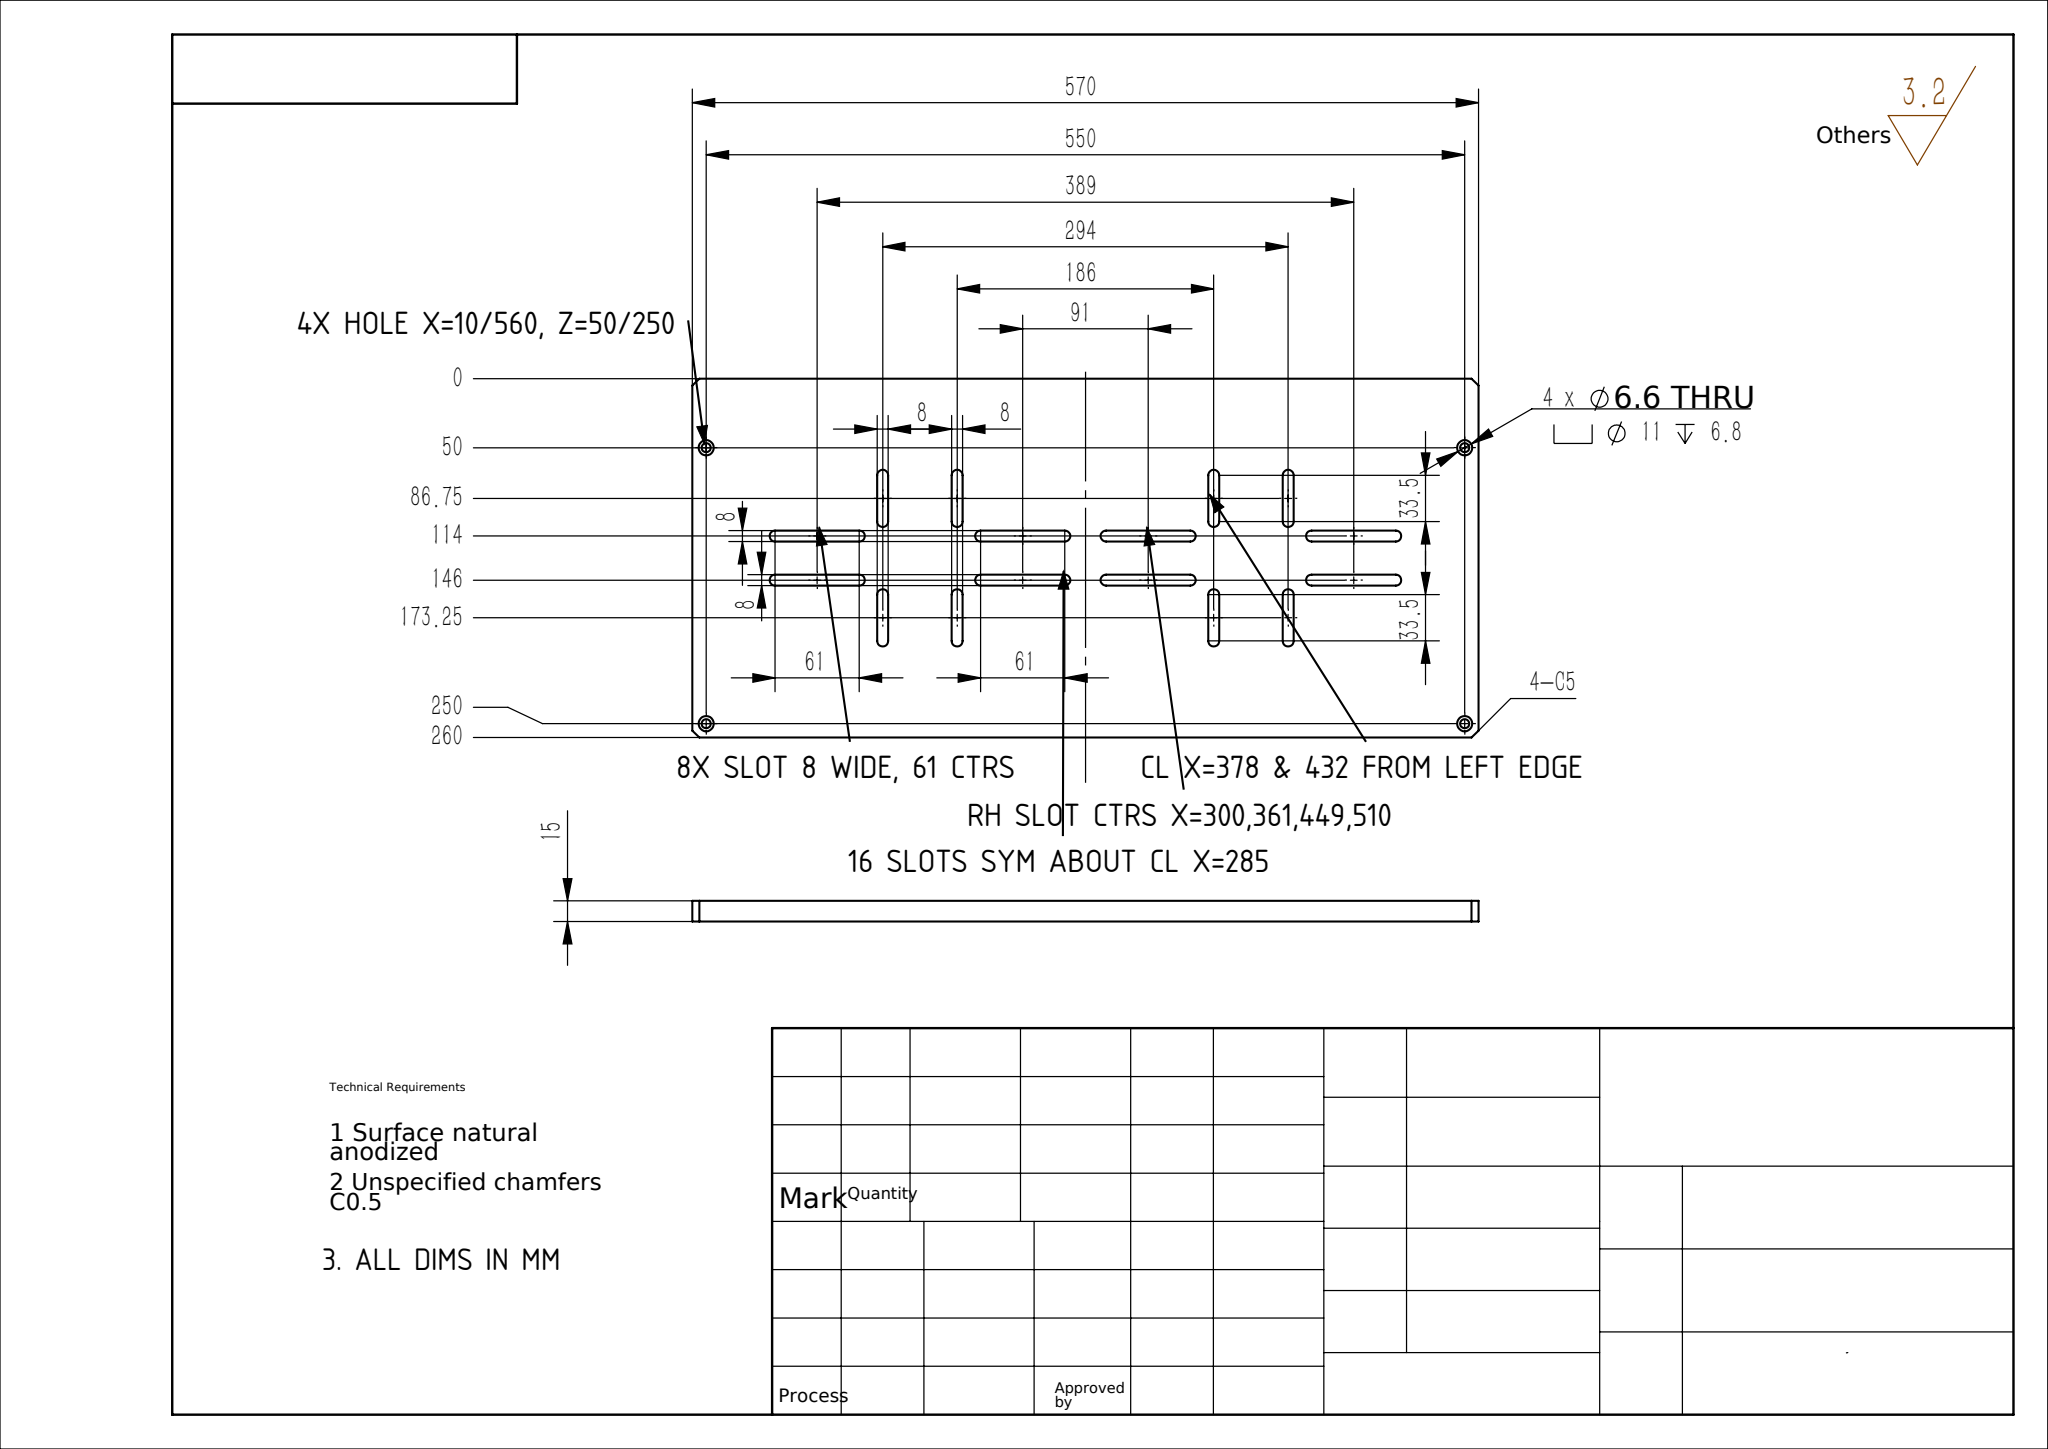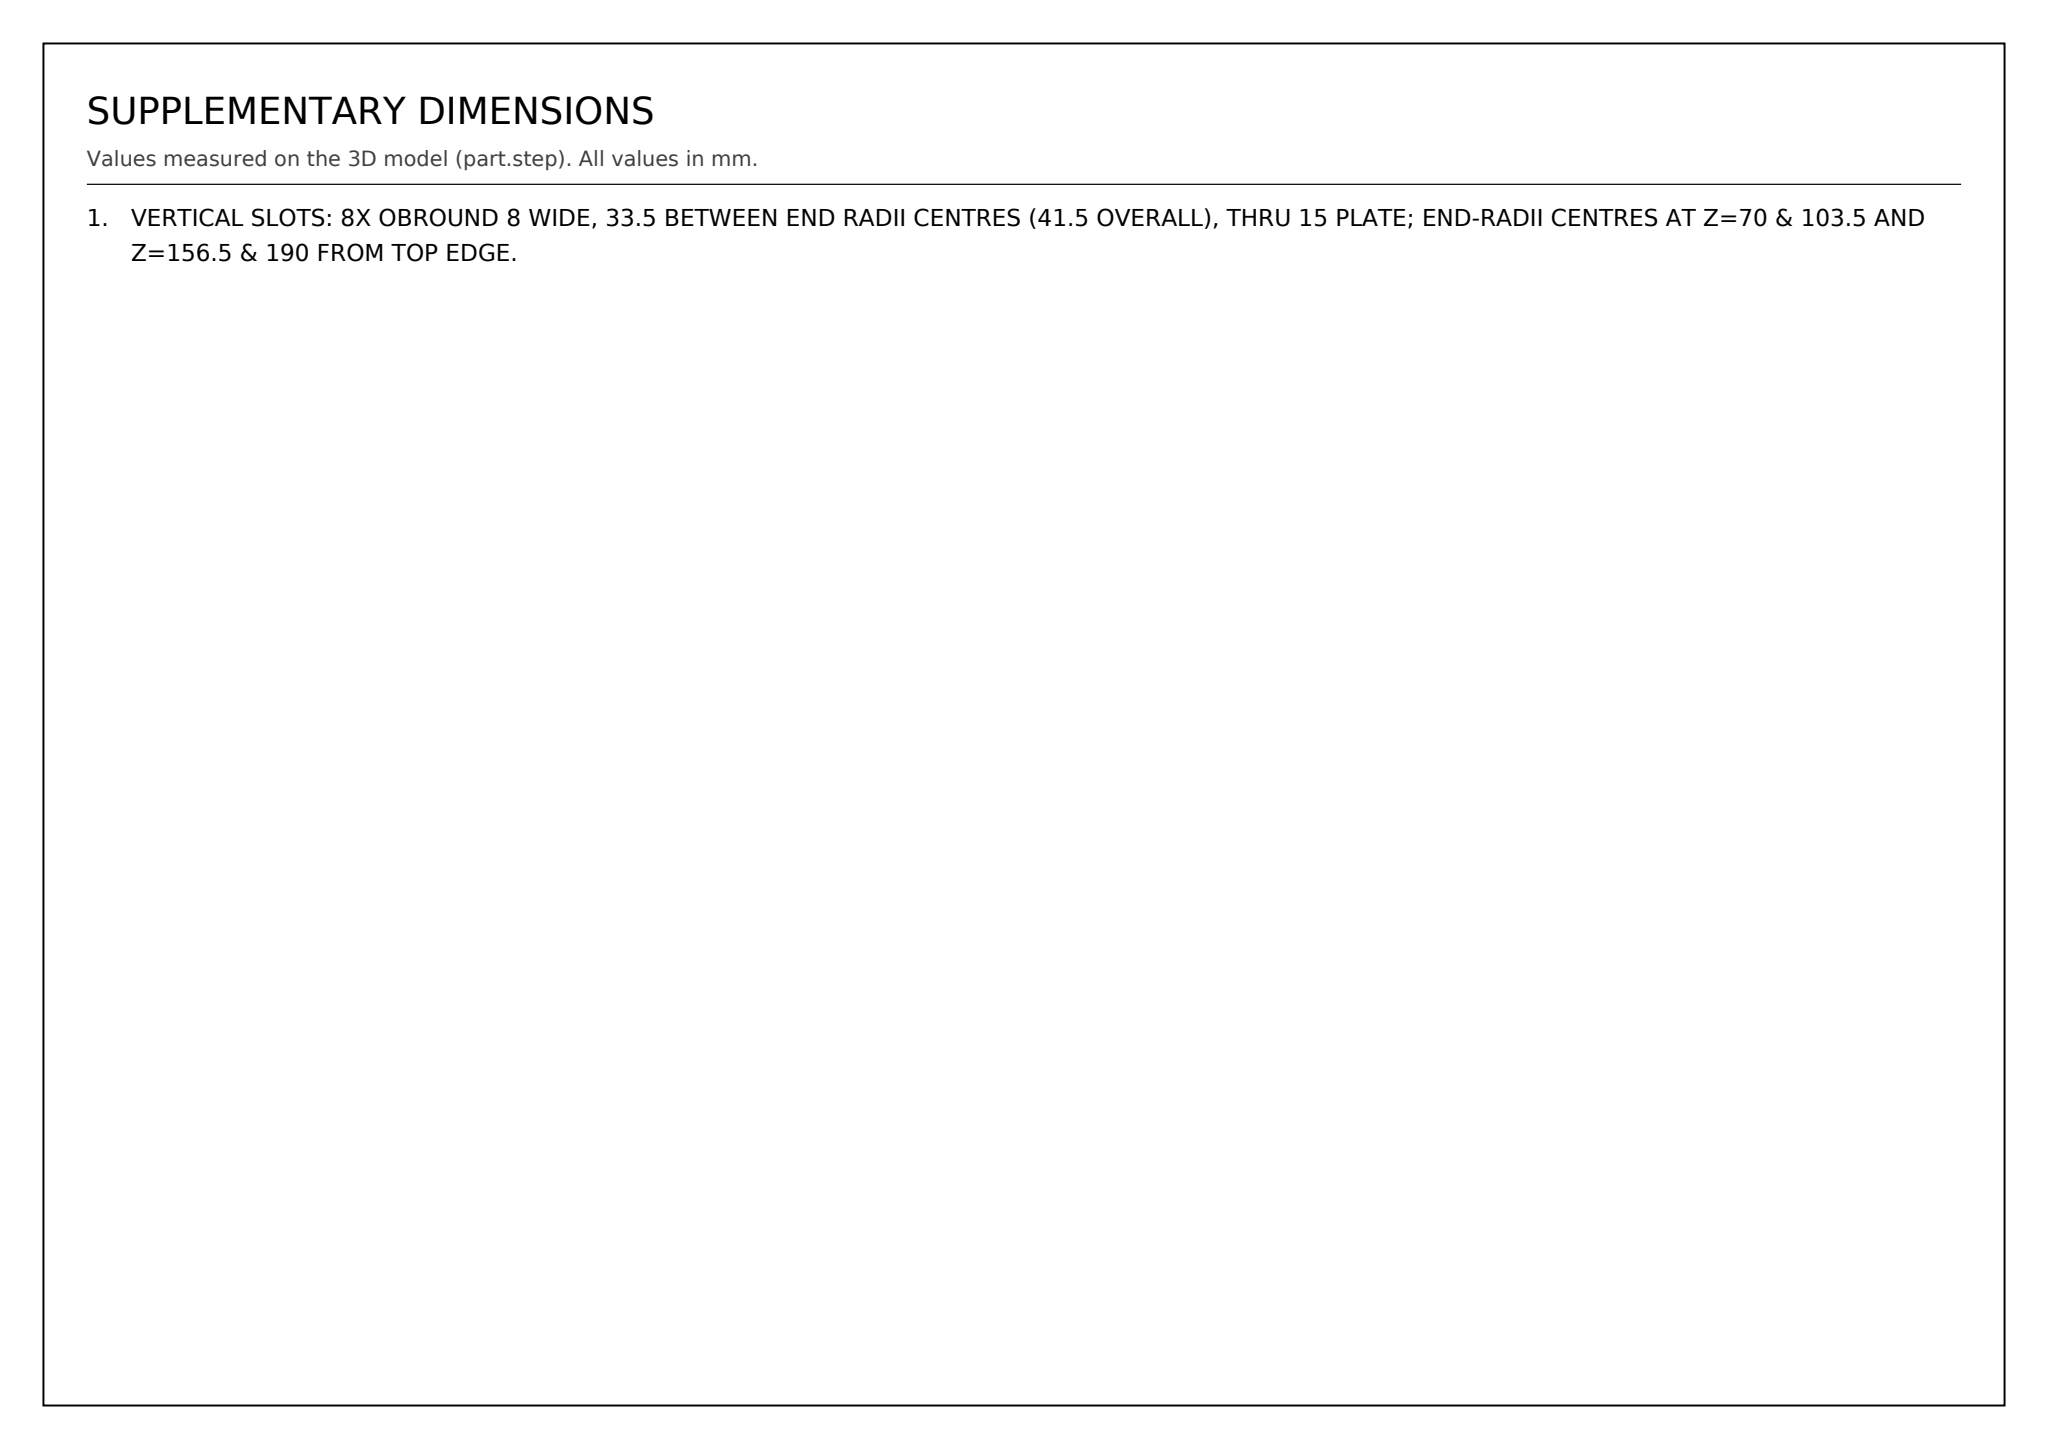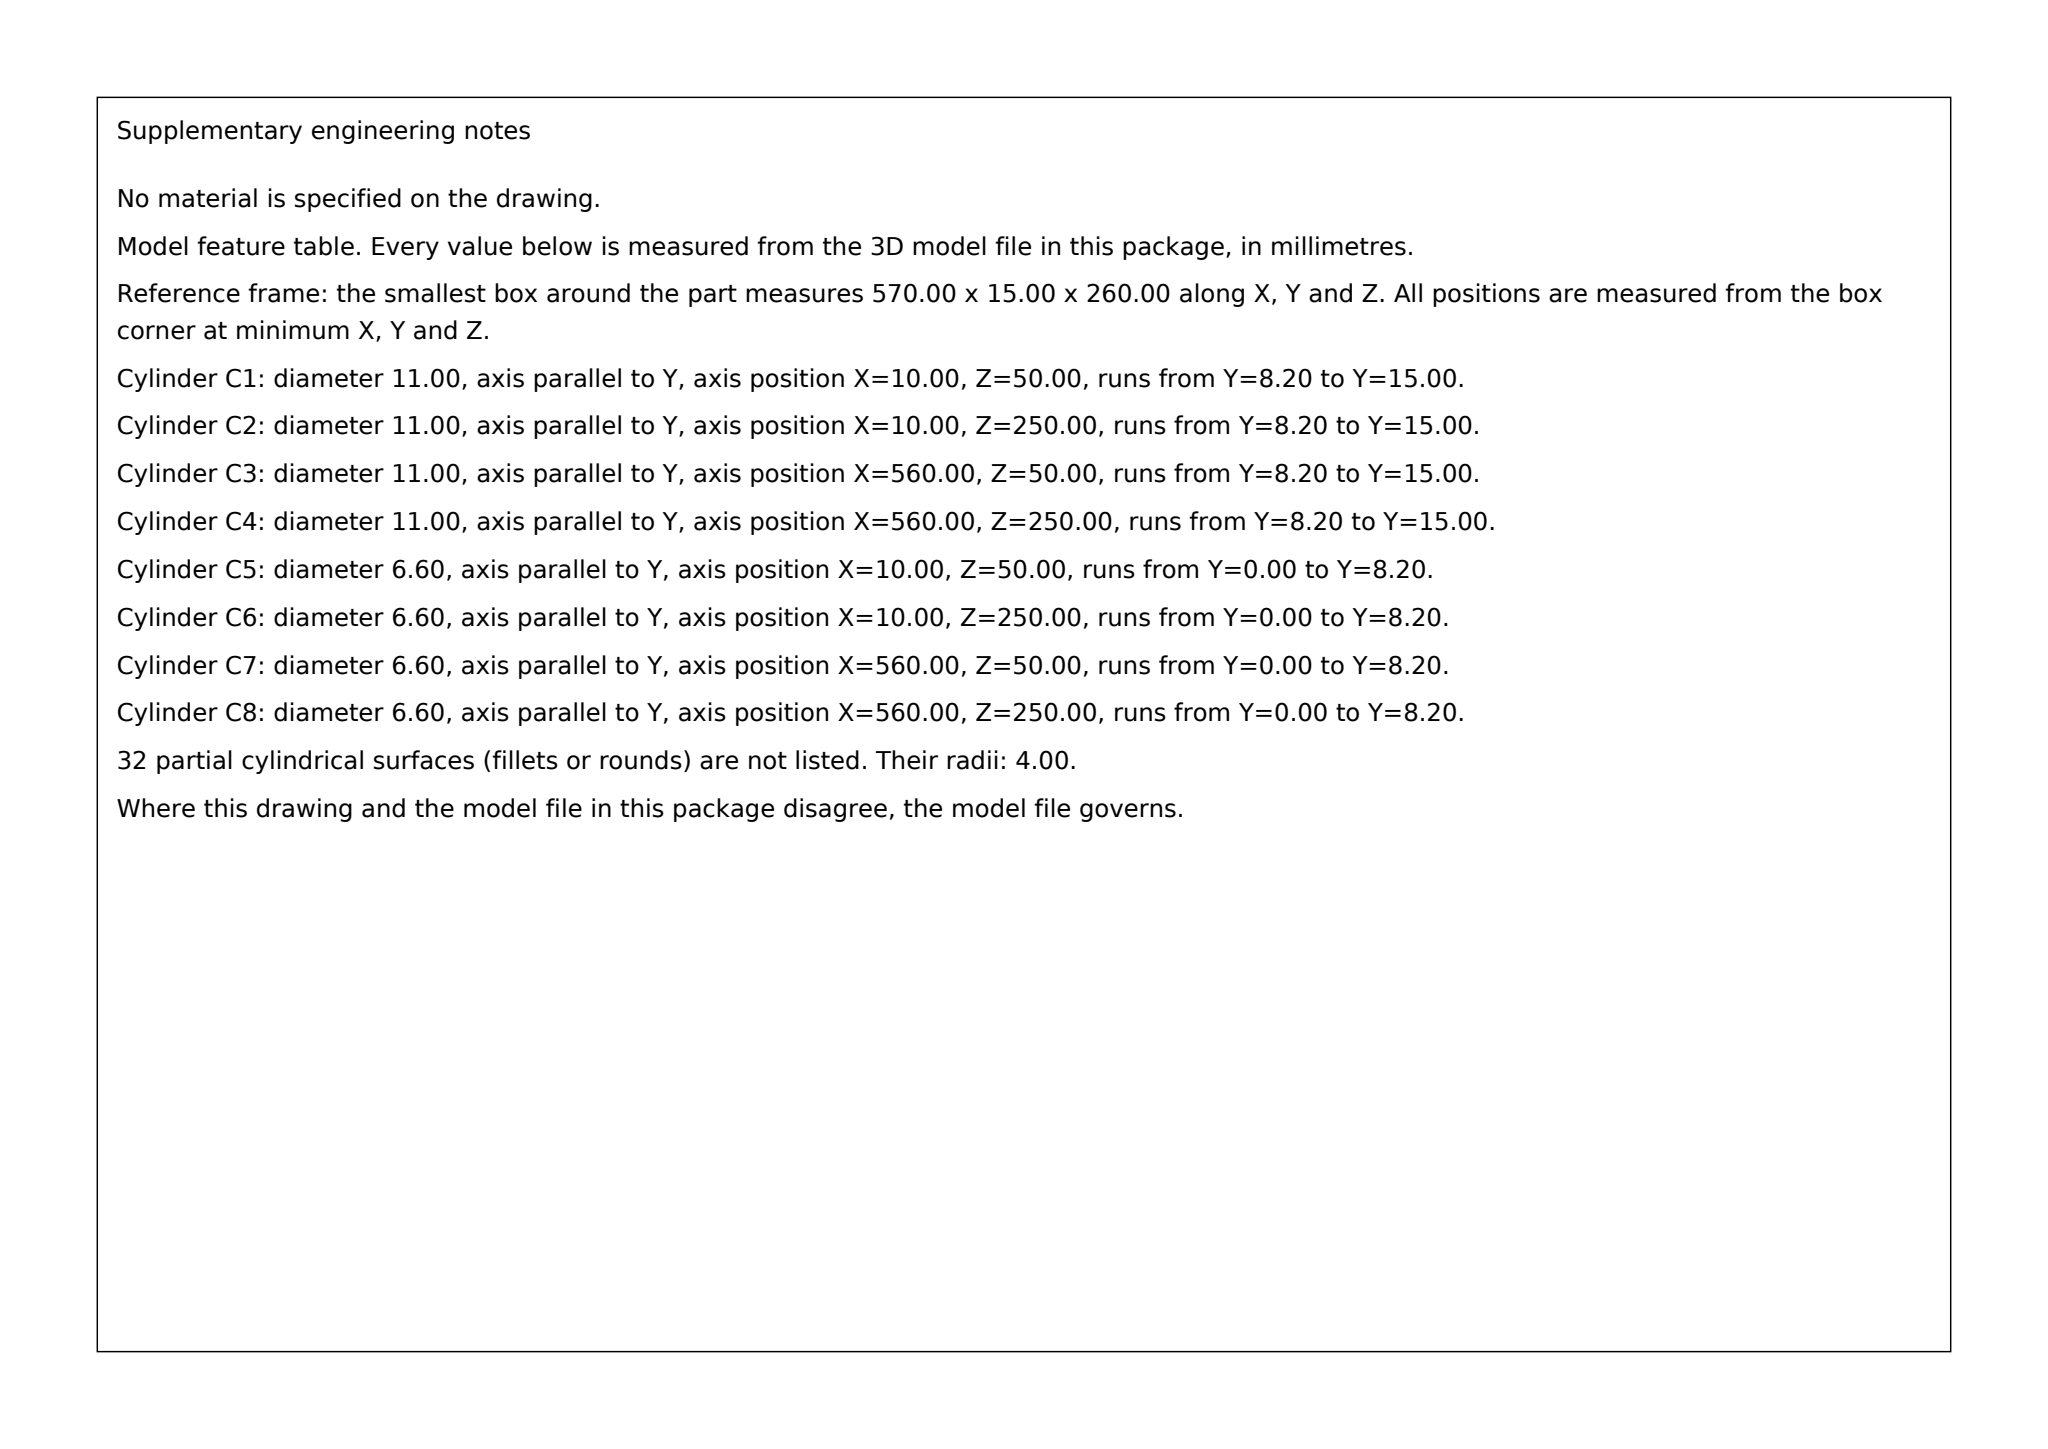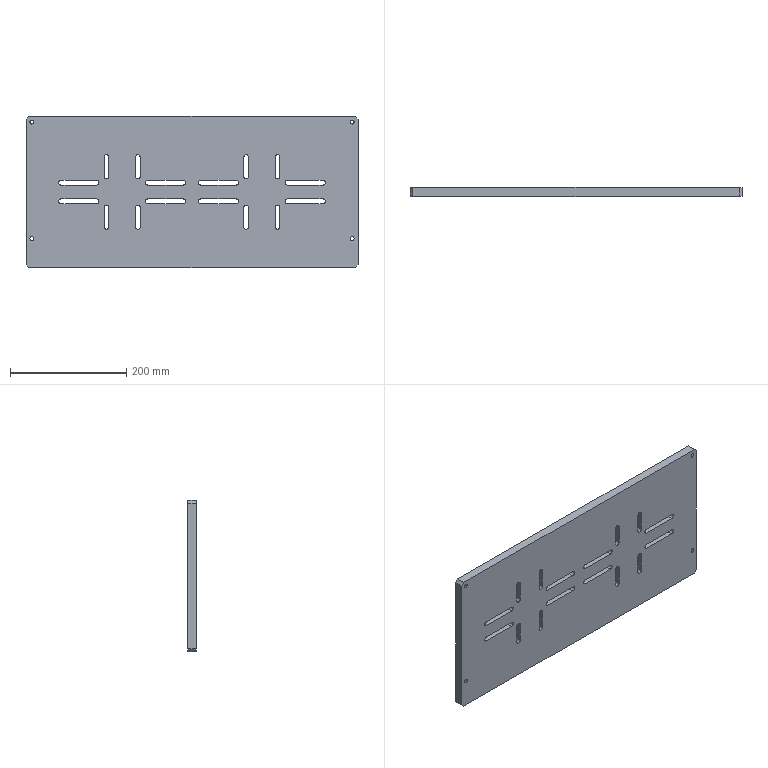Part | SolidWorks | mm | 1 solid | 102 faces | box 570 x 15 x 260 mm | volume 2115759 mm3 | cylinder 56 | plane 46 | commonest cylinder face diameters 8 x40 11 x8 6.6 x8
Drawing notes:
ALL DIMS IN MM | from the solid: STEP model length unit = mm (geometry data n/a otherwise)
HORIZONTAL SLOTS: 8X OBROUND 8 WIDE, 61 BETWEEN END RADII CENTRES (69 OVERALL), THRU 15 PLATE; END-RADII CENTRES AT Z=114 AND Z=146 FROM TOP EDGE. | from the solid: cylinders dia 8.0 axis y len 15.0 at (60,114),(121,114),(60,146),(121,146) etc.; axis_planes z=110/118 and z=142/150; bbox y=15
VERTICAL SLOTS: 8X OBROUND 8 WIDE, 33.5 BETWEEN END RADII CENTRES (41.5 OVERALL), THRU 15 PLATE; END-RADII CENTRES AT Z=70 & 103.5 AND Z=156.5 & 190 FROM TOP EDGE. | from the solid: cylinders dia 8.0 axis y len 15.0 at z=70,103.5,156.5,190 for x=138,192,378,432; axis_planes x=134/142,188/196,374/382,428/436
RIGHT-HAND HORIZONTAL SLOTS: END-RADII CENTRES AT X=300, 361, 449 AND 510 FROM LEFT EDGE. | from the solid: cylinders dia 8.0 axis y at x=300,361,449,510 with z=114 and 146
RIGHT-HAND VERTICAL SLOTS: CENTRELINES AT X=378 AND X=432 FROM LEFT EDGE. | from the solid: cylinders dia 8.0 axis y at x=378 and 432 (z=70,103.5,156.5,190); axis_planes x=374/382 and 428/436
SLOT PATTERN: 16 SLOTS TOTAL (8 HORIZONTAL + 8 VERTICAL), SYMMETRIC ABOUT PLATE CENTRELINE X=285. | from the solid: cylinder list: 32 dia 8.0 holes forming 16 slots; x pairs 60/510, 121/449, 209/361, 270/300, 138/432, 192/378 each sum to 570 (bbox x=570)
4X Ø6.6 THRU, CBORE Ø11 DEPTH 6.8; HOLE CENTRES AT X=10 AND X=560 FROM LEFT EDGE, Z=50 AND Z=250 FROM TOP EDGE. | from the solid: cylinders dia 6.6 len 8.2 and dia 11.0 len 6.8 at (10,50),(10,250),(560,50),(560,250); 8.2+6.8=15 = bbox y thickness
build123d program:
from build123d import *

# Parameters (mm, degrees)
SKETCH_1_W                = 330
SKETCH_1_H                = 260
EXTRUDE_1_DEPTH           = 15
CUT_EXTRUDE_1_DEPTH       = 211.594
CUT_EXTRUDE_2_DEPTH       = 211.594
SKETCH_6_W                = 285
SKETCH_6_H                = 260
EXTRUDE_2_DEPTH           = 15
HOLE_WIZARD_1_D           = 6.6
HOLE_WIZARD_1_CBORE_D     = 11
HOLE_WIZARD_1_CBORE_DEPTH = 6.8
CHAMFER_1_SIZE            = 5


with BuildPart() as part:
    # Sketch 1 → Extrude 1 (new body)
    with BuildSketch(Plane(origin=(0, 0, 0), x_dir=(1, 0, 0), z_dir=(0, 1, 0))):
        Rectangle(SKETCH_1_W, SKETCH_1_H)
    extrude(amount=EXTRUDE_1_DEPTH)

    # Sketch 2 → Cut-Extrude 1 (cut, through all)
    with BuildSketch(Plane(origin=(0, 15, 0), x_dir=(1, 0, 0), z_dir=(0, 1, 0))):
        with BuildLine():
            Line((23, -60), (23, -26.5))
            ThreePointArc((23, -26.5), (27, -22.5), (31, -26.5))
            Line((31, -26.5), (31, -60))
            ThreePointArc((31, -60), (27, -64), (23, -60))
        make_face()
        with BuildLine():
            Line((-23, -60), (-23, -26.5))
            ThreePointArc((-23, -26.5), (-27, -22.5), (-31, -26.5))
            Line((-31, -26.5), (-31, -60))
            ThreePointArc((-31, -60), (-27, -64), (-23, -60))
        make_face()
        with BuildLine():
            Line((-44, -20), (-105, -20))
            ThreePointArc((-105, -20), (-109, -16), (-105, -12))
            Line((-105, -12), (-44, -12))
            ThreePointArc((-44, -12), (-40, -16), (-44, -20))
        make_face()
        with BuildLine():
            Line((-44, 20), (-105, 20))
            ThreePointArc((-105, 20), (-109, 16), (-105, 12))
            Line((-105, 12), (-44, 12))
            ThreePointArc((-44, 12), (-40, 16), (-44, 20))
        make_face()
        with BuildLine():
            Line((-23, 60), (-23, 26.5))
            ThreePointArc((-23, 26.5), (-27, 22.5), (-31, 26.5))
            Line((-31, 26.5), (-31, 60))
            ThreePointArc((-31, 60), (-27, 64), (-23, 60))
        make_face()
        with BuildLine():
            Line((23, 60), (23, 26.5))
            ThreePointArc((23, 26.5), (27, 22.5), (31, 26.5))
            Line((31, 26.5), (31, 60))
            ThreePointArc((31, 60), (27, 64), (23, 60))
        make_face()
        with BuildLine():
            Line((44, 20), (105, 20))
            ThreePointArc((105, 20), (109, 16), (105, 12))
            Line((105, 12), (44, 12))
            ThreePointArc((44, 12), (40, 16), (44, 20))
        make_face()
        with BuildLine():
            Line((44, -20), (105, -20))
            ThreePointArc((105, -20), (109, -16), (105, -12))
            Line((105, -12), (44, -12))
            ThreePointArc((44, -12), (40, -16), (44, -20))
        make_face()
    cut_extrude_1 = extrude(amount=-CUT_EXTRUDE_1_DEPTH, mode=Mode.SUBTRACT)

    # Sketch 3 → Cut-Extrude 2 (cut, through all)
    with BuildSketch(Plane(origin=(0, 15, 0), x_dir=(1, 0, 0), z_dir=(0, 1, 0))):
        Polygon((120, 143.676), (181.892, 143.676), (181.892, -162.375), (120, -162.375), align=None)
    extrude(amount=-CUT_EXTRUDE_2_DEPTH, mode=Mode.SUBTRACT)

    # Sketch 6 → Extrude 2 (add)
    with BuildSketch(Plane(origin=(0, 15, 0), x_dir=(1, 0, 0), z_dir=(0, 1, 0))):
        with Locations((262.5, 0)):
            Rectangle(SKETCH_6_W, SKETCH_6_H)
    extrude(amount=-EXTRUDE_2_DEPTH)

    # Mirror 1: Cut-Extrude 1 across plane
    add(cut_extrude_1.mirror(Plane.ZY.offset(-120)), mode=Mode.SUBTRACT)

    # Hole Wizard 1 (through all)
    with Locations(Plane(origin=(0, 15, 0), x_dir=(1, 0, 0), z_dir=(0, 1, 0))):
        with Locations((-155, 80), (395, 80), (395, -120), (-155, -120)):
            CounterBoreHole(HOLE_WIZARD_1_D / 2, HOLE_WIZARD_1_CBORE_D / 2, HOLE_WIZARD_1_CBORE_DEPTH)

    # Chamfer 1
    chamfer_1_edges = [part.edges().sort_by_distance(p)[0] for p in [
        (405, 7.5, -130),
        (405, 7.5, 130),
        (-165, 7.5, 130),
        (-165, 7.5, -130),
    ]]
    chamfer(chamfer_1_edges, length=CHAMFER_1_SIZE)


solid = part.part